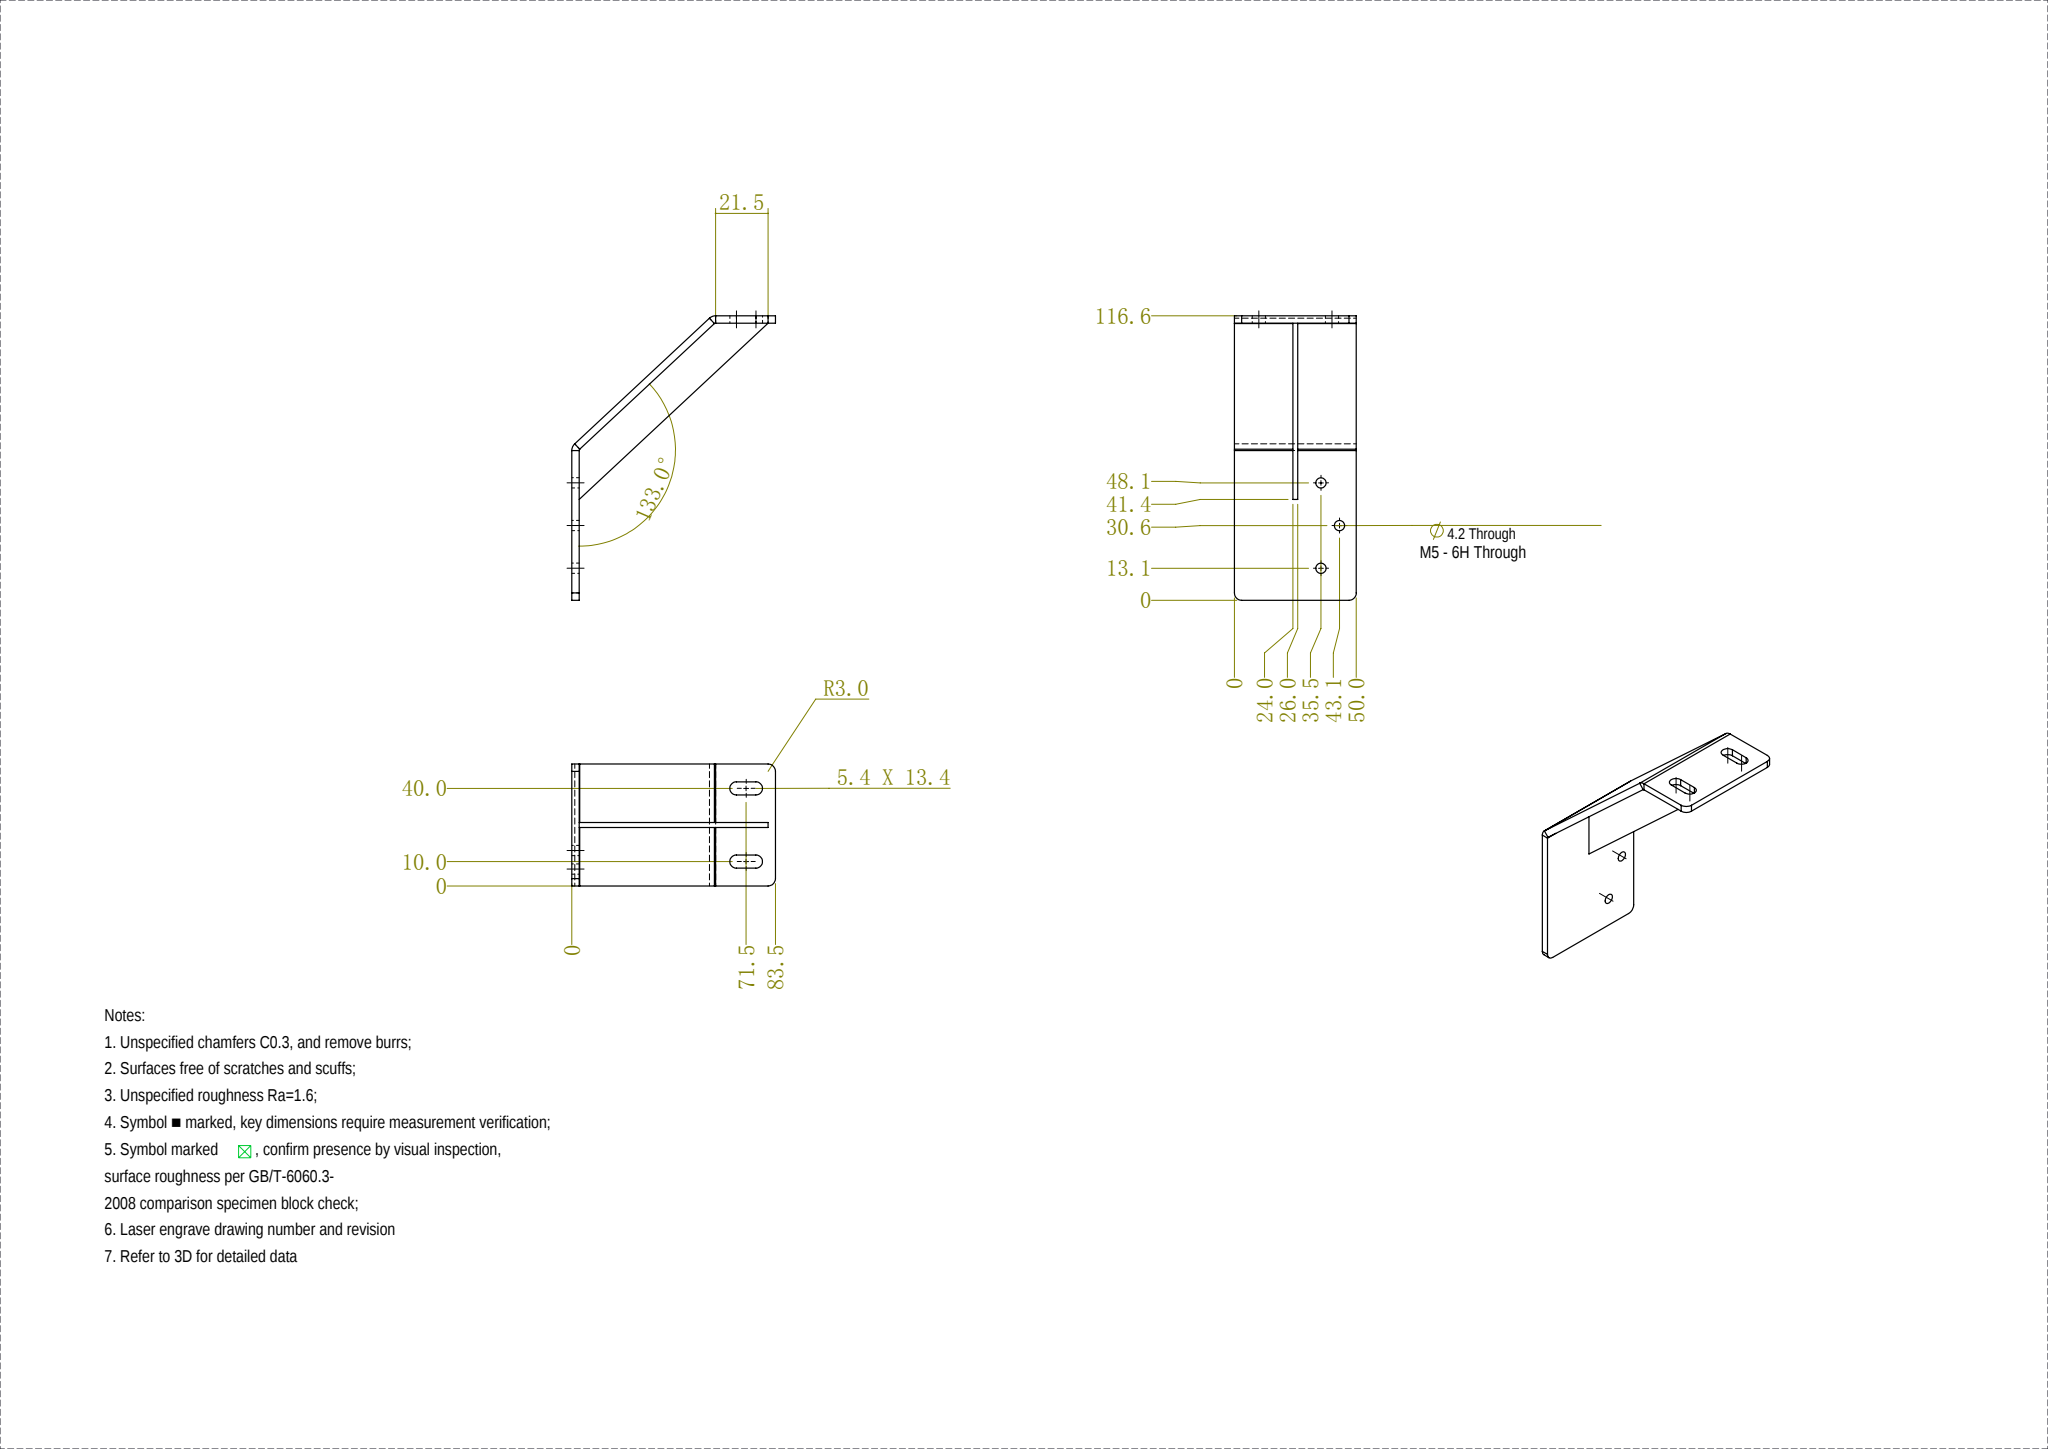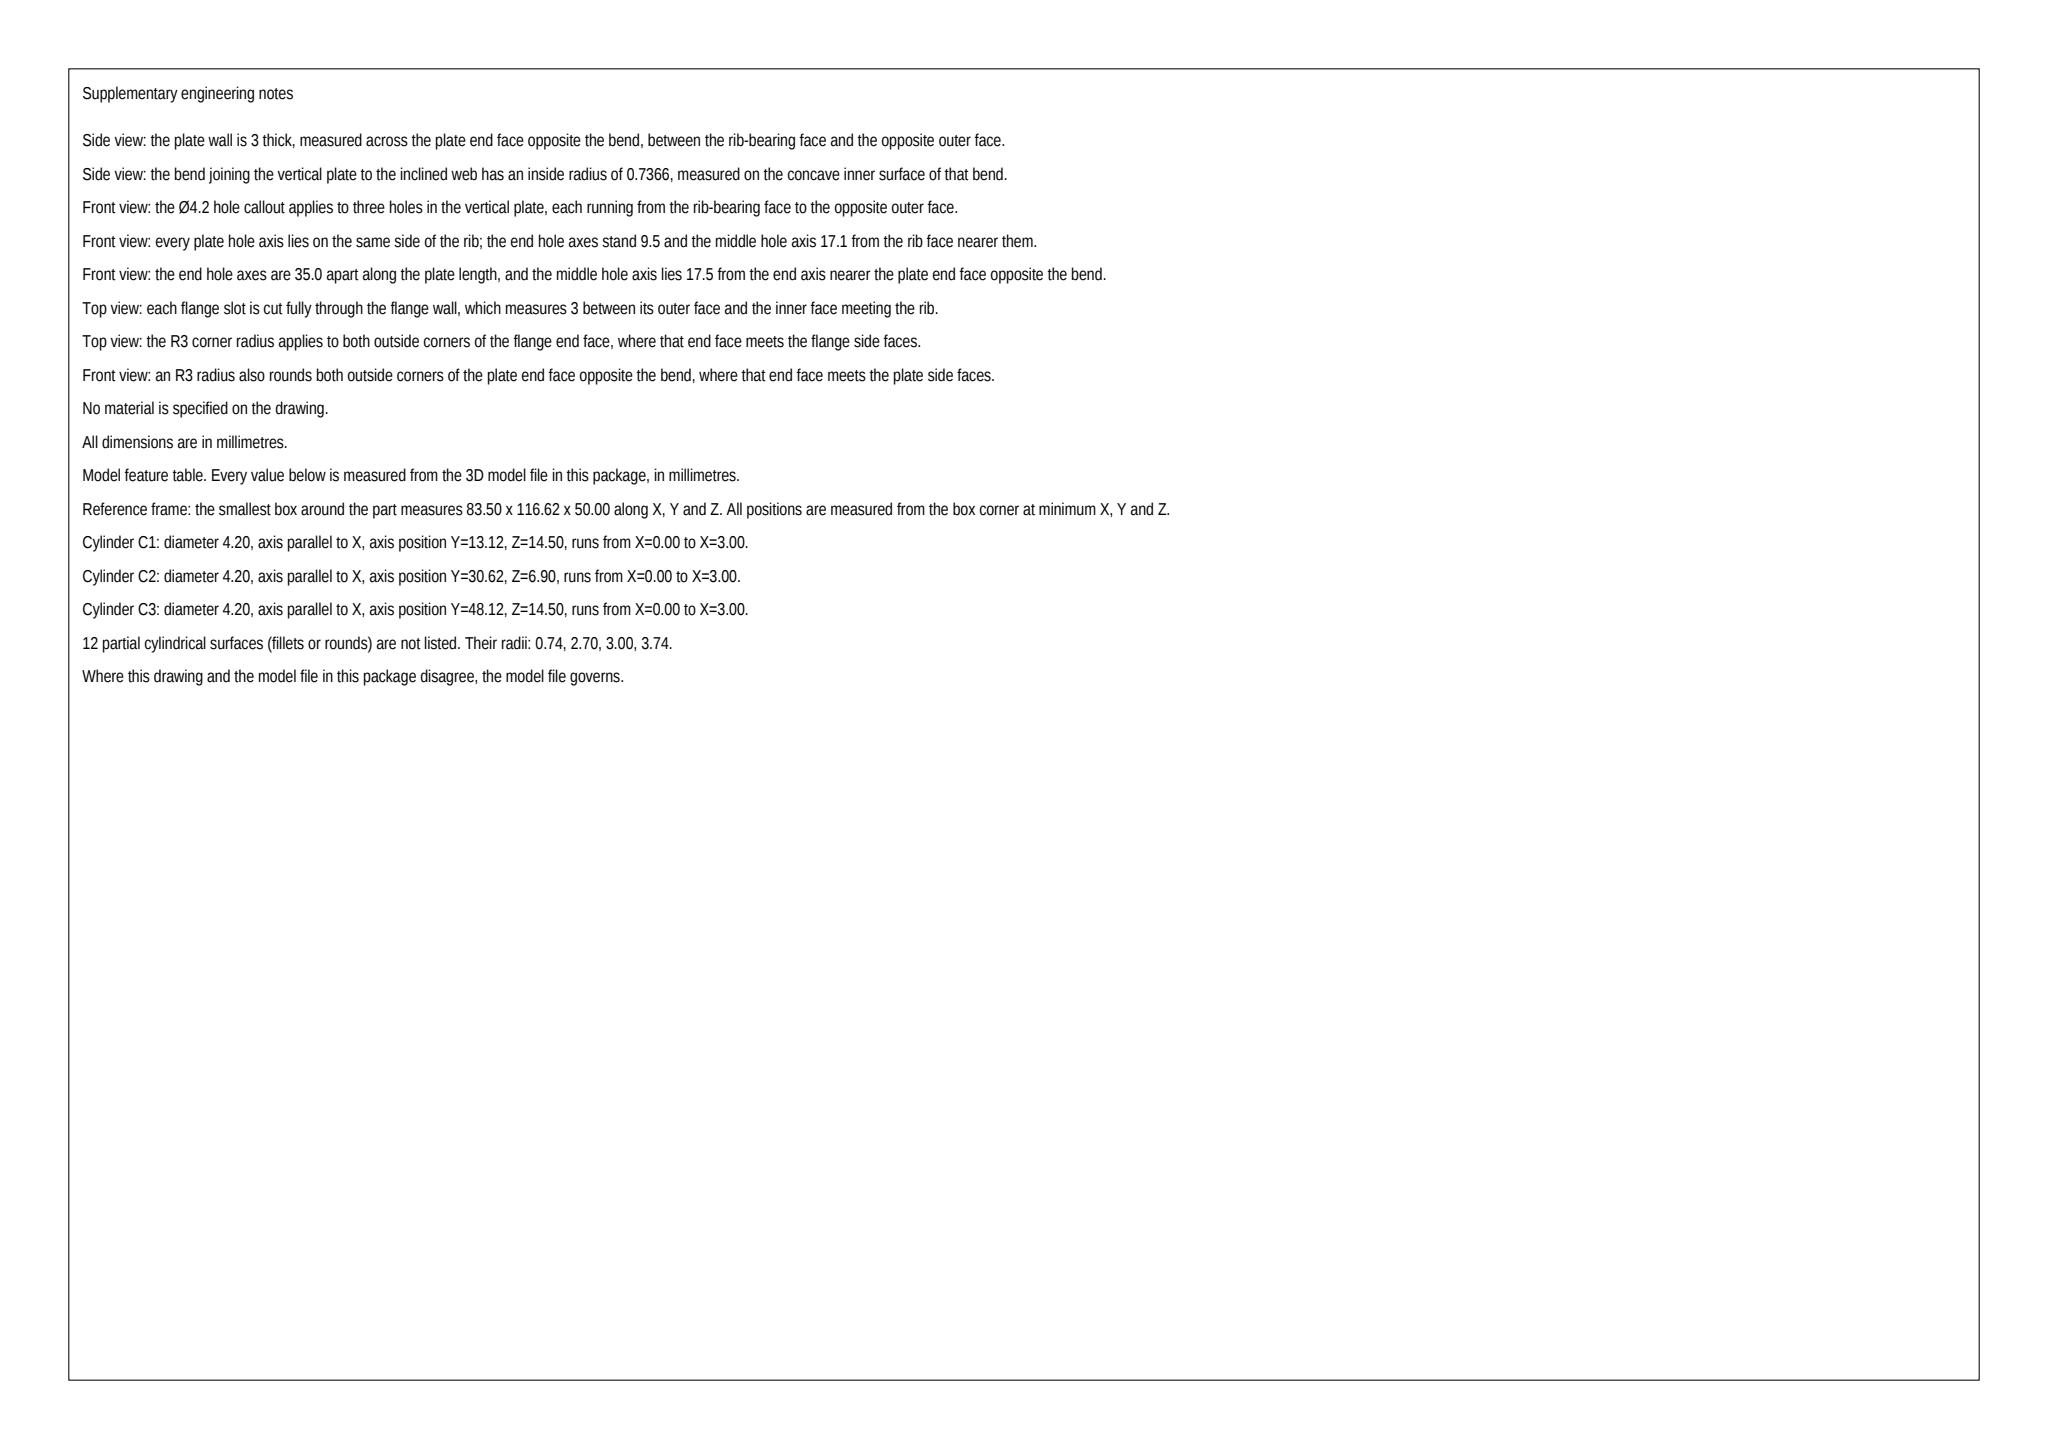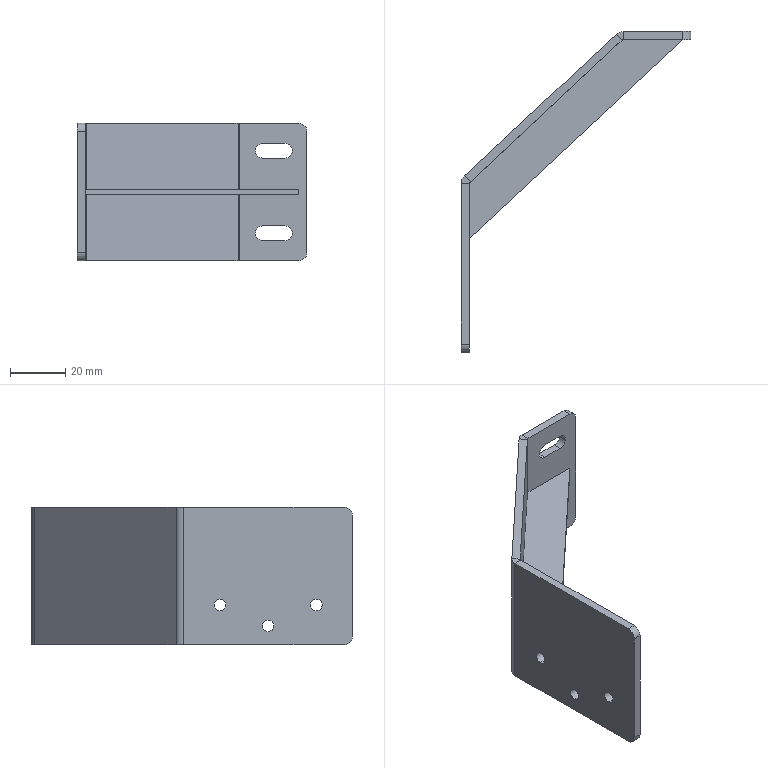Part | SolidWorks | mm | 1 solid | 48 faces | box 83.5 x 116.62 x 50 mm | volume 26902 mm3 | plane 26 | cylinder 22 | commonest cylinder face diameters 4.2 x6 5.4 x6 1.473 x4 6 x4 7.473 x2